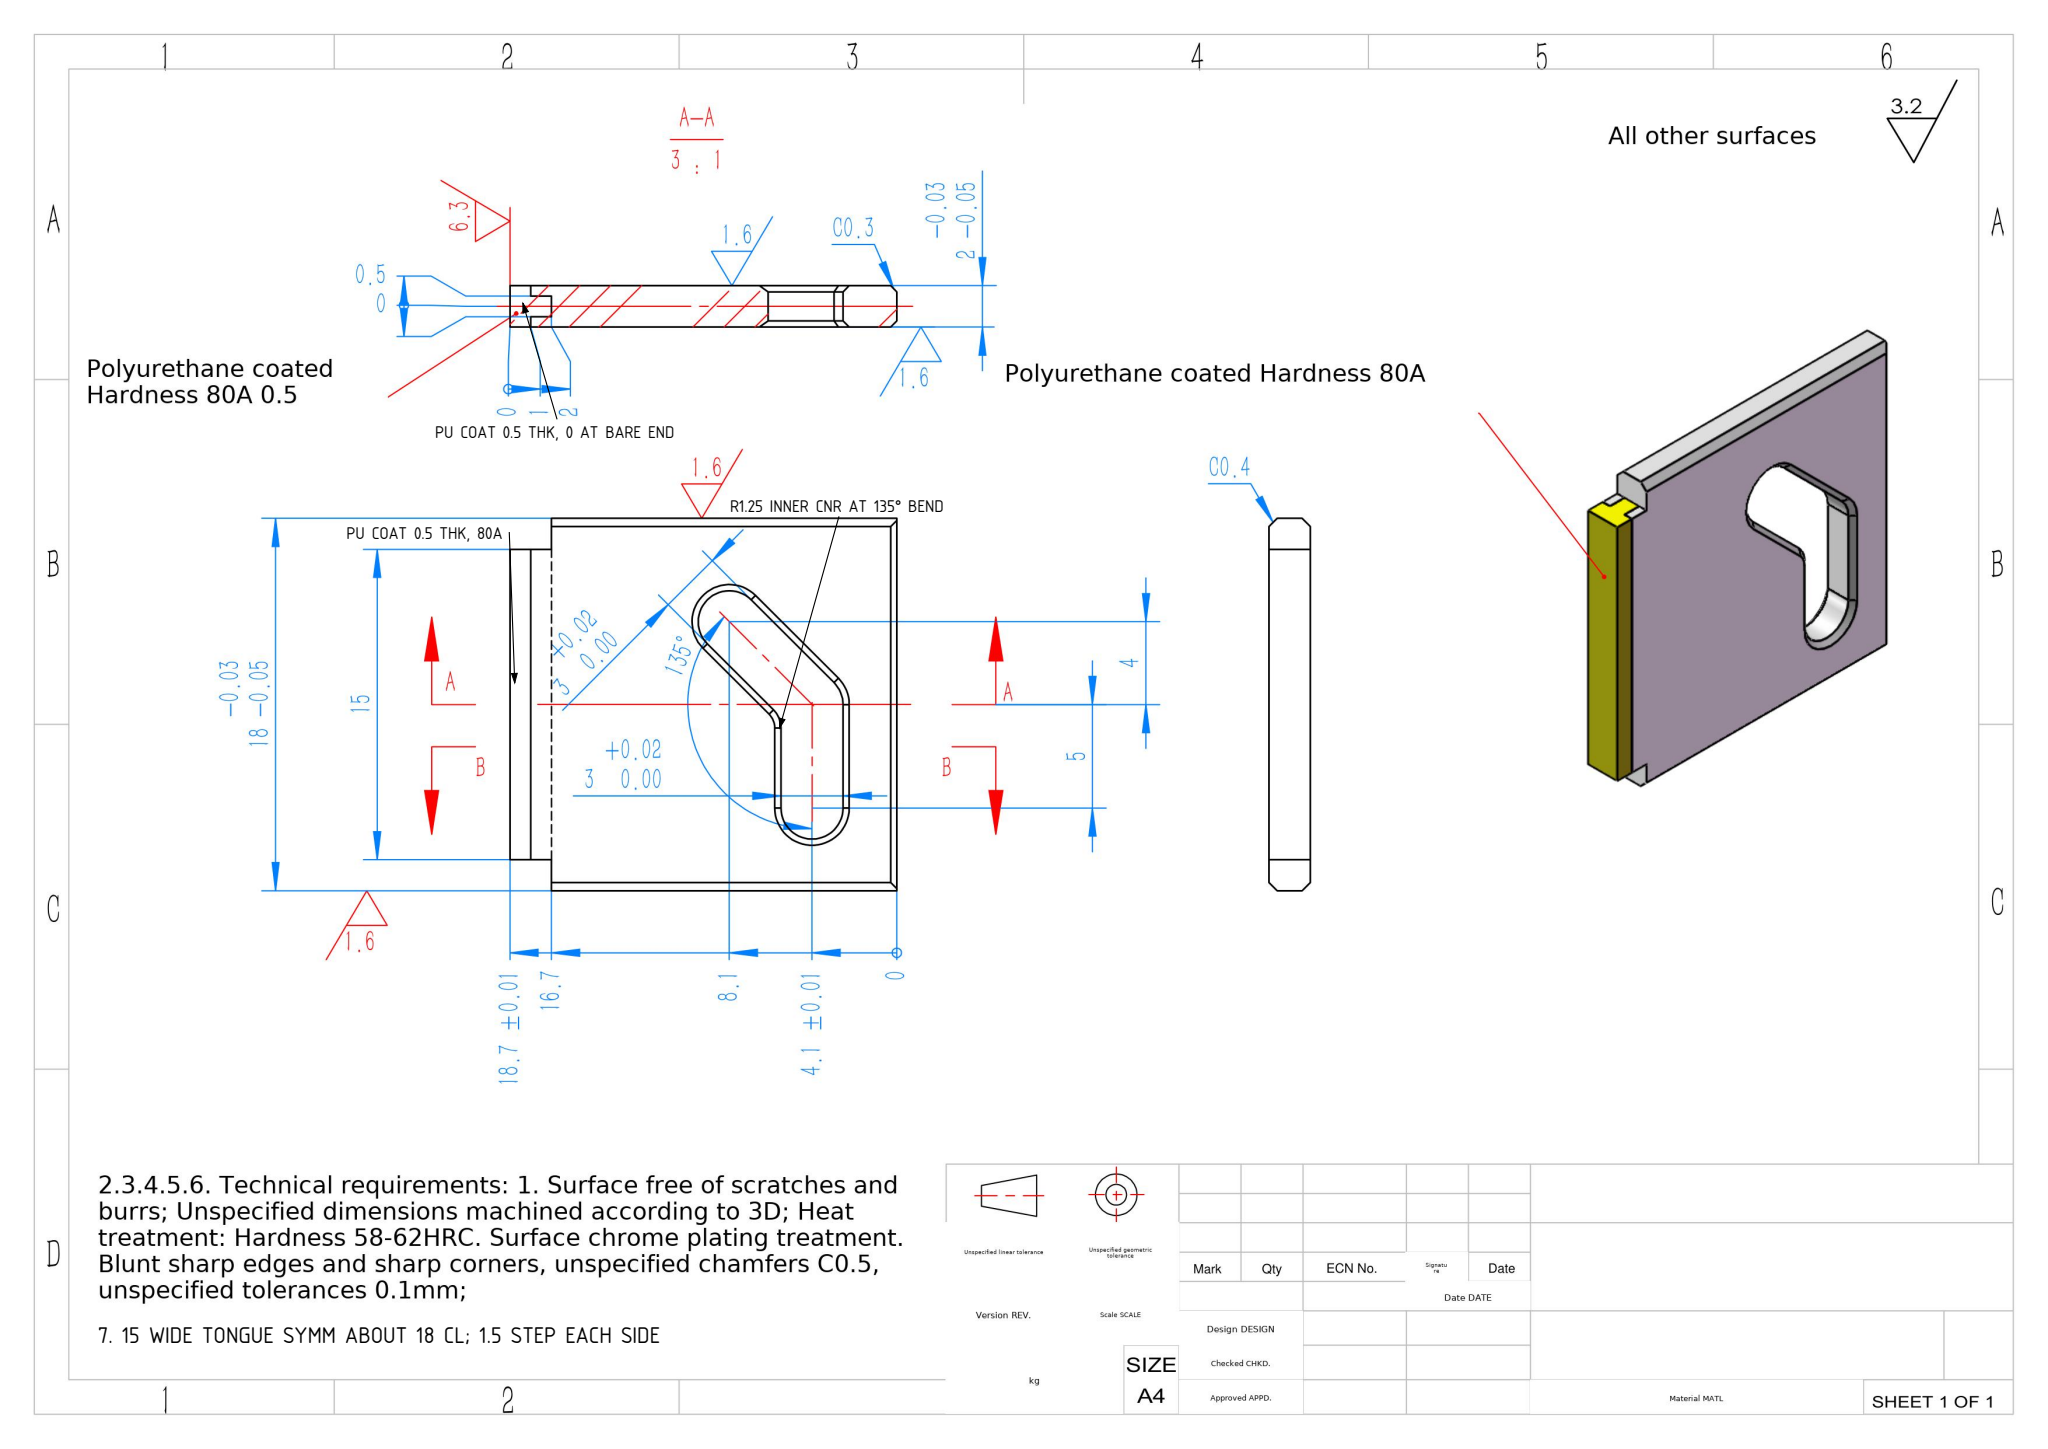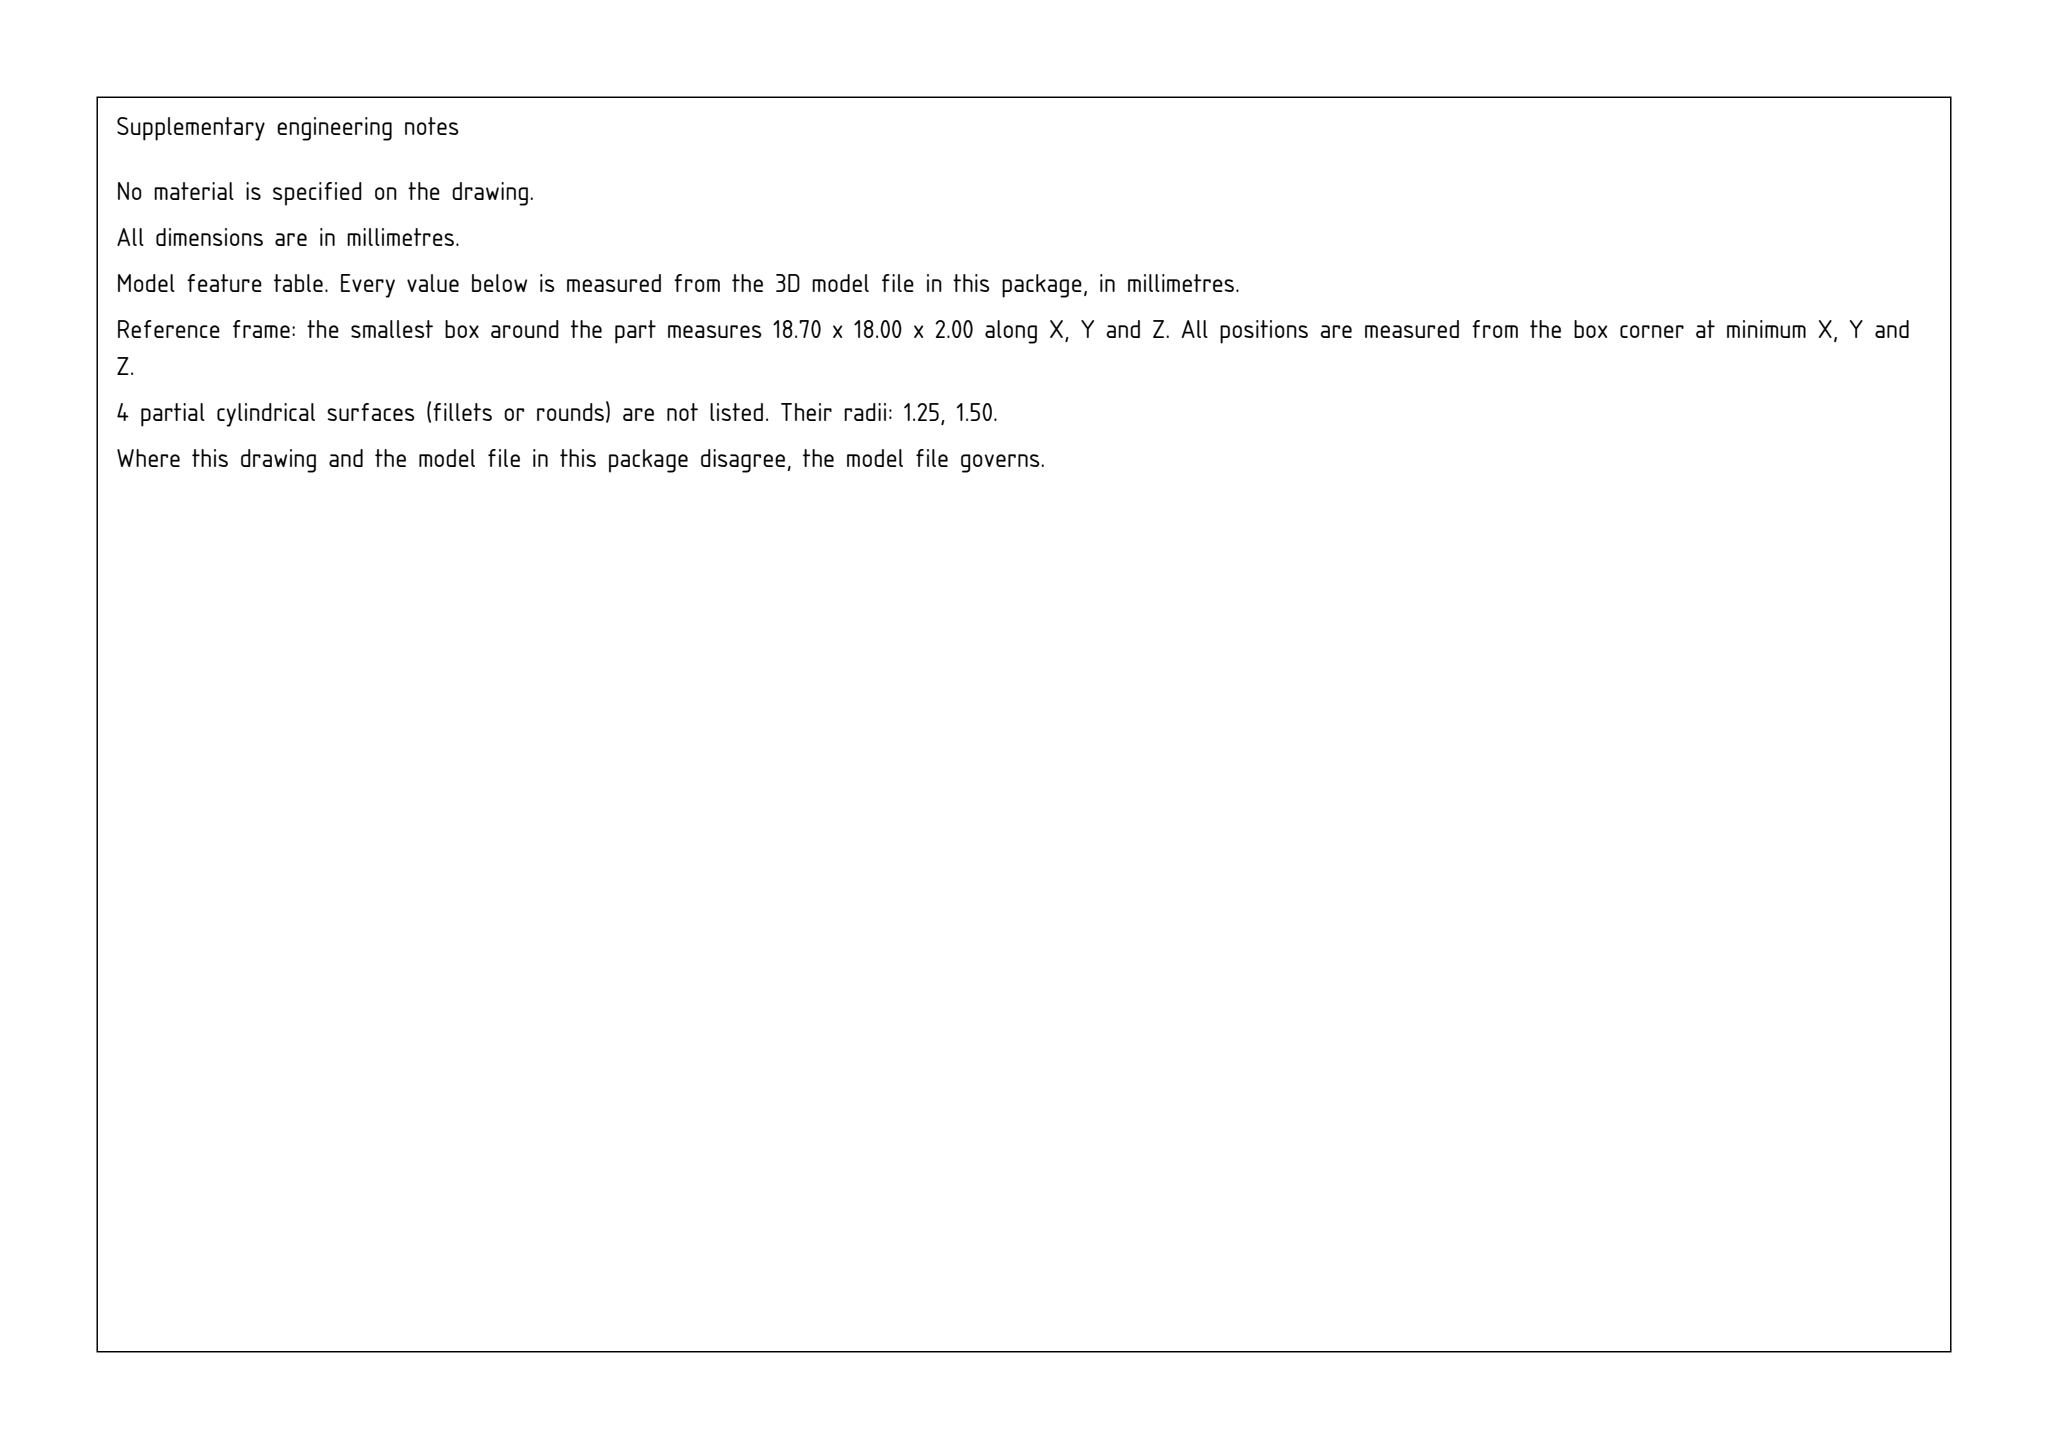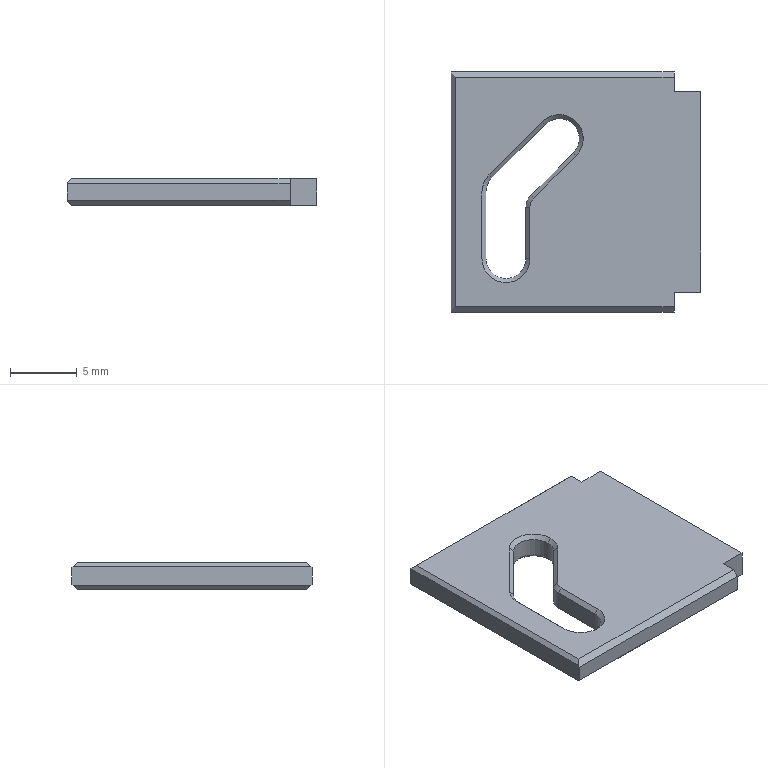Part | SolidWorks | mm | 1 solid | 42 faces | box 18.7 x 18 x 2 mm | volume 573 mm3 | plane 28 | cone 9 | cylinder 5 | commonest cylinder face diameters 3 x4 2.5 x1
Drawing notes:
R1.25 SLOT INNER CNR AT 135° BEND; CTR 6.9 FROM 0 ORD, 7.9 FROM BTM | from the solid: convex arc dia 2.5 (R1.25), axis z at x=6.9, y=7.9, 45 deg, z 0.3-1.7
15 WIDE TONGUE SYMM ABOUT 18 CL; 1.5 STEP EACH SIDE | from the solid: x=18.7 face y 1.5-16.5 (15 wide); x=16.7 faces y 0-1.5 and 16.5-18.0 in 18 overall
PU COATING 0.5 THK, HARDNESS 80A, ON 18.7 END FACE OF TONGUE | from the solid: coated face = plane x=18.7, extent y 1.5-16.5, z 0-2, area 30; 0.5 = coat thk from note
SECT A-A 0.5/0 = PU COAT 0.5 THK, 0 AT BARE END FACE X18.7 | from the solid: stacked 0.5/0 on leader at tongue end; only x=18.7 end face (area 30) is coated
build123d program:
from build123d import *

# Parameters (mm, degrees)
SKETCH1_W           = 17.7
SKETCH1_H           = 18
BOSS_EXTRUDE1_DEPTH = 1
CUT_EXTRUDE1_DEPTH  = 10
CUT_EXTRUDE2_DEPTH  = 10
FILLET1_R           = 1.25
CHAMFER1_SIZE       = 0.4
CHAMFER3_SIZE       = 0.3
CHAMFER9_SIZE       = 0.4
SKETCH8_W           = 2
SKETCH8_H           = 1
CUT_EXTRUDE4_DEPTH  = 21.083
SKETCH10_W          = 1
SKETCH10_H          = 1.5
CUT_EXTRUDE5_DEPTH  = 10
BOSS_EXTRUDE2_DEPTH = 15


with BuildPart() as part:
    # Sketch1 → Boss-Extrude1 (new, symmetric)
    with BuildSketch(Plane.XY):
        Rectangle(SKETCH1_W, SKETCH1_H)
    extrude(amount=BOSS_EXTRUDE1_DEPTH, both=True)

    # Sketch2 → Cut-Extrude1 (cut)
    with BuildSketch(Plane.XY.offset(1)):
        with BuildLine():
            Line((-5.811, 1.061), (-1.811, 5.061))
            ThreePointArc((-1.811, 5.061), (0.3107, 5.061), (0.3107, 2.939))
            Line((0.3107, 2.939), (-3.689, -1.061))
            ThreePointArc((-3.689, -1.061), (-5.811, -1.061), (-5.811, 1.061))
        make_face()
    extrude(amount=-CUT_EXTRUDE1_DEPTH, mode=Mode.SUBTRACT)

    # Sketch3 → Cut-Extrude2 (cut)
    with BuildSketch(Plane(origin=(0, 0, -1), x_dir=(-1, 0, 0), z_dir=(0, 0, -1))):
        with BuildLine():
            Line((6.25, 0), (3.25, -0.6213))
            Line((3.25, -0.6213), (3.25, -5))
            ThreePointArc((3.25, -5), (4.75, -6.5), (6.25, -5))
            Line((6.25, -5), (6.25, 0))
        make_face()
    extrude(amount=-CUT_EXTRUDE2_DEPTH, mode=Mode.SUBTRACT)

    # Fillet1
    fillet1_edges = [part.edges().sort_by_distance(p)[0] for p in [
        (-3.25, -0.6213, 0),
    ]]
    fillet(fillet1_edges, radius=FILLET1_R)

    # Chamfer1
    chamfer1_edges = [part.edges().sort_by_distance(p)[0] for p in [
        (0, 9, 1),
        (0, 9, -1),
        (0, -9, -1),
    ]]
    chamfer(chamfer1_edges, length=CHAMFER1_SIZE)

    # Chamfer3
    chamfer3_edges = [part.edges().sort_by_distance(p)[0] for p in [
        (0.3107, 5.061, -1),
        (-3.811, 3.061, -1),
        (-6.136, 0.574, -1),
        (-6.136, 0.574, 1),
        (0.3107, 5.061, 1),
        (-3.811, 3.061, 1),
        (-4.75, -6.5, 1),
        (-6.25, -2.5, 1),
        (-3.25, -3.07, -1),
        (-4.75, -6.5, -1),
        (-6.25, -2.5, -1),
        (-3.25, -3.07, 1),
        (-1.287, 1.342, -1),
        (-3.155, -0.6607, -1),
        (-1.287, 1.342, 1),
        (-3.155, -0.6607, 1),
        (-8.85, 0, -1),
        (-8.85, -0.2, 1),
    ]]
    chamfer(chamfer3_edges, length=CHAMFER3_SIZE)

    # Chamfer9
    chamfer9_edges = [part.edges().sort_by_distance(p)[0] for p in [
        (0.15, -9, 1),
    ]]
    chamfer(chamfer9_edges, length=CHAMFER9_SIZE)

    # Sketch8 → Cut-Extrude4 (cut, through all)
    with BuildSketch(Plane(origin=(0, 9, 0), x_dir=(1, 0, 0), z_dir=(0, 1, 0))):
        with Locations((8.85, 0)):
            Rectangle(SKETCH8_W, SKETCH8_H)
    extrude(amount=-CUT_EXTRUDE4_DEPTH, mode=Mode.SUBTRACT)

    # Sketch10 → Cut-Extrude5 (cut)
    with BuildSketch(Plane.XY.offset(1)):
        with Locations((8.35, -8.25)):
            Rectangle(SKETCH10_W, SKETCH10_H)
        with Locations((8.35, 8.25)):
            Rectangle(SKETCH10_W, SKETCH10_H)
    extrude(amount=-CUT_EXTRUDE5_DEPTH, mode=Mode.SUBTRACT)


with BuildPart() as body_2:
    # Sketch12 → Boss-Extrude2 (new body)
    with BuildSketch(Plane(origin=(0, 7.5, 0), x_dir=(1, 0, 0), z_dir=(0, 1, 0))):
        Polygon((7.85, -0.5), (7.85, 0.5), (8.85, 0.5), (8.85, 1), (9.85, 1), (9.85, -1), (8.85, -1), (8.85, -0.5), align=None)
    extrude(amount=-BOSS_EXTRUDE2_DEPTH)

    # Combine-RayDong-Repair: union part
    add(part.part)


solid = body_2.part